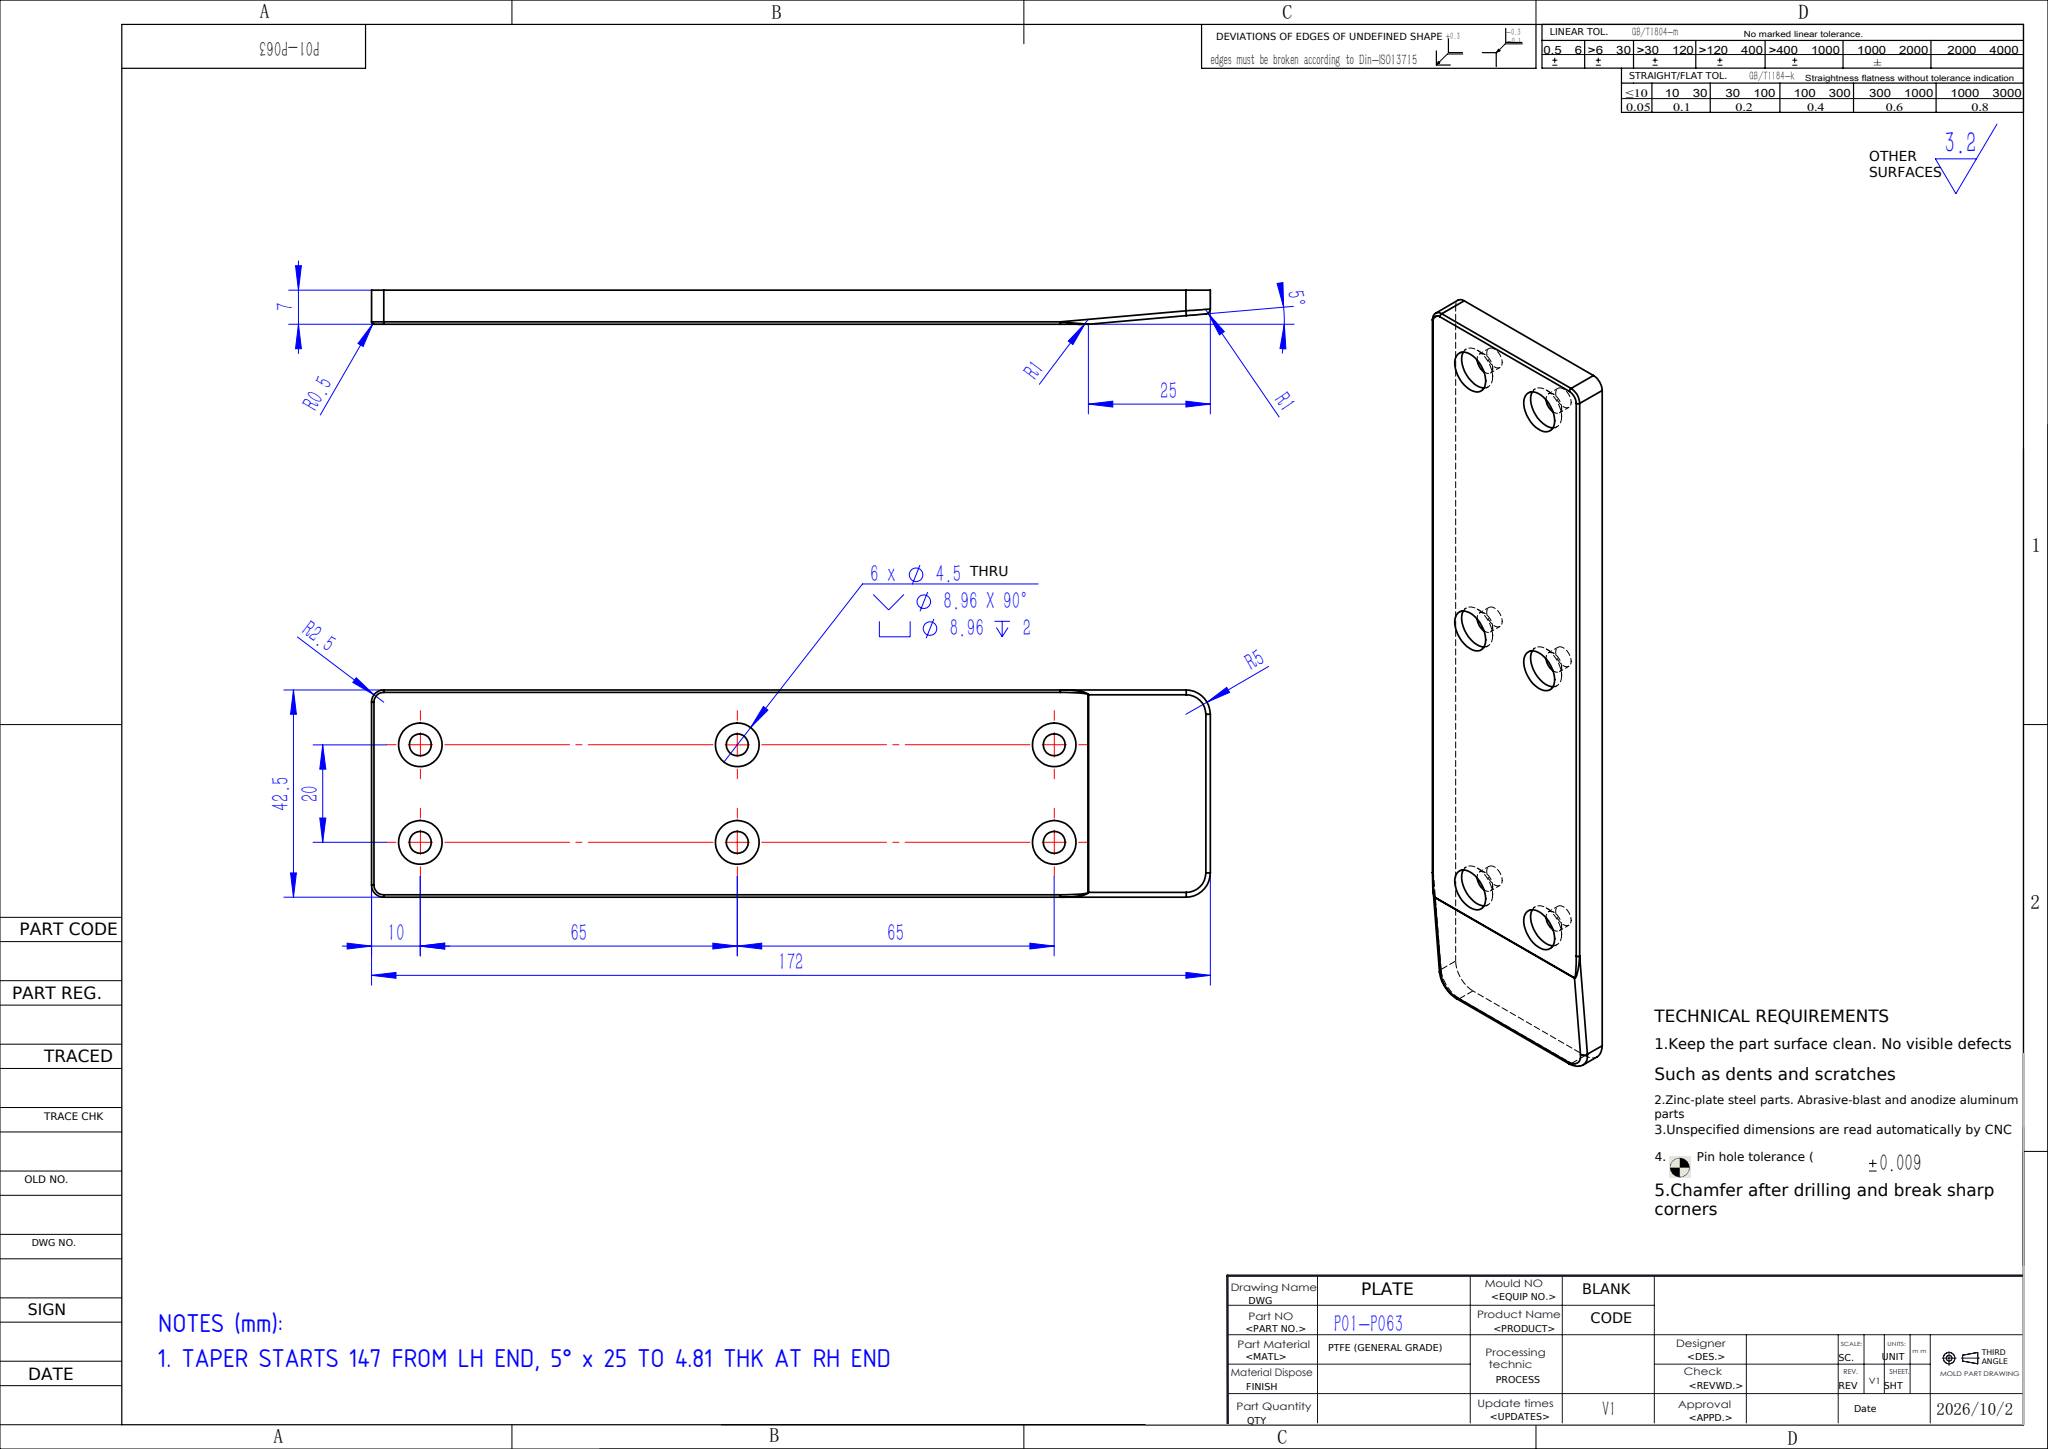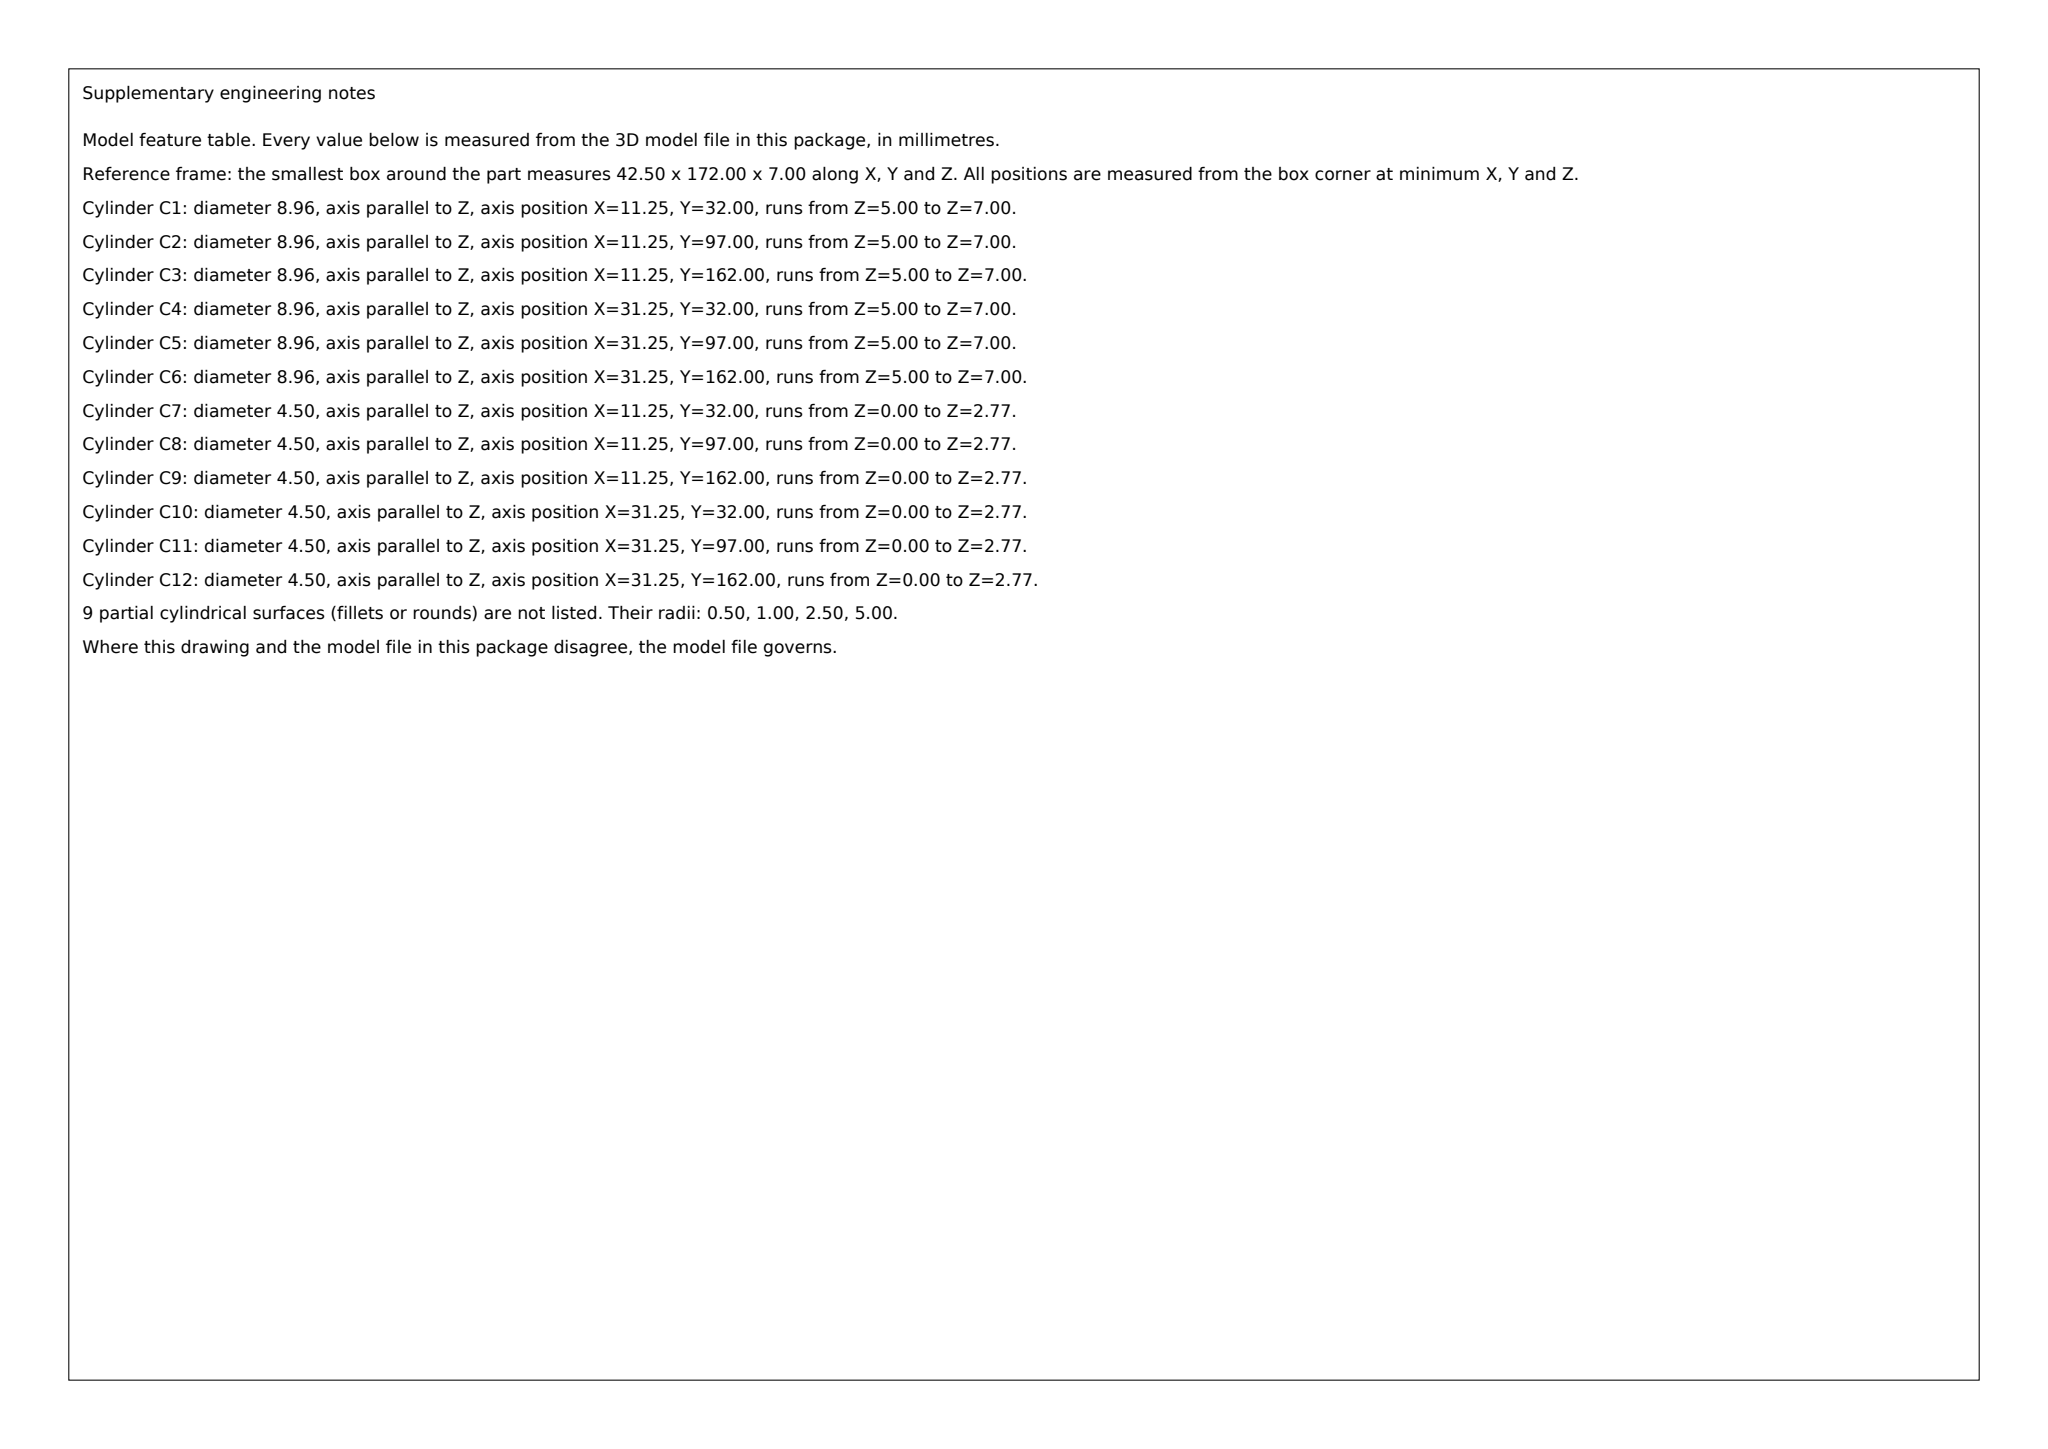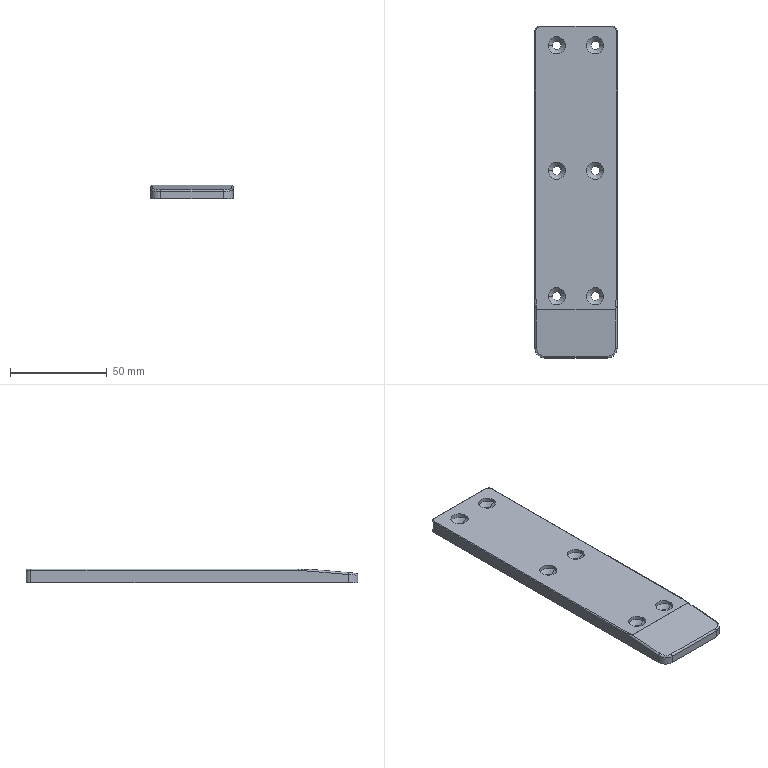Part | SolidWorks | mm | 1 solid | 62 faces | box 42.5 x 172 x 7 mm | volume 48387 mm3 | cylinder 35 | cone 12 | plane 7 | spline 6 | torus 2 | commonest cylinder face diameters 8.96 x12 4.5 x12 2 x4 1 x3 5 x2 10 x2
Drawing notes:
TAPER STARTS 147 FROM LH END, 5° x 25 TO 4.81 THK AT RH END | from the solid: R1 fillet axis at y=25.04 on top face z=7, plate y=0..172 (172-25=147); z planes 0 and 7, 7-25*tan5=4.813